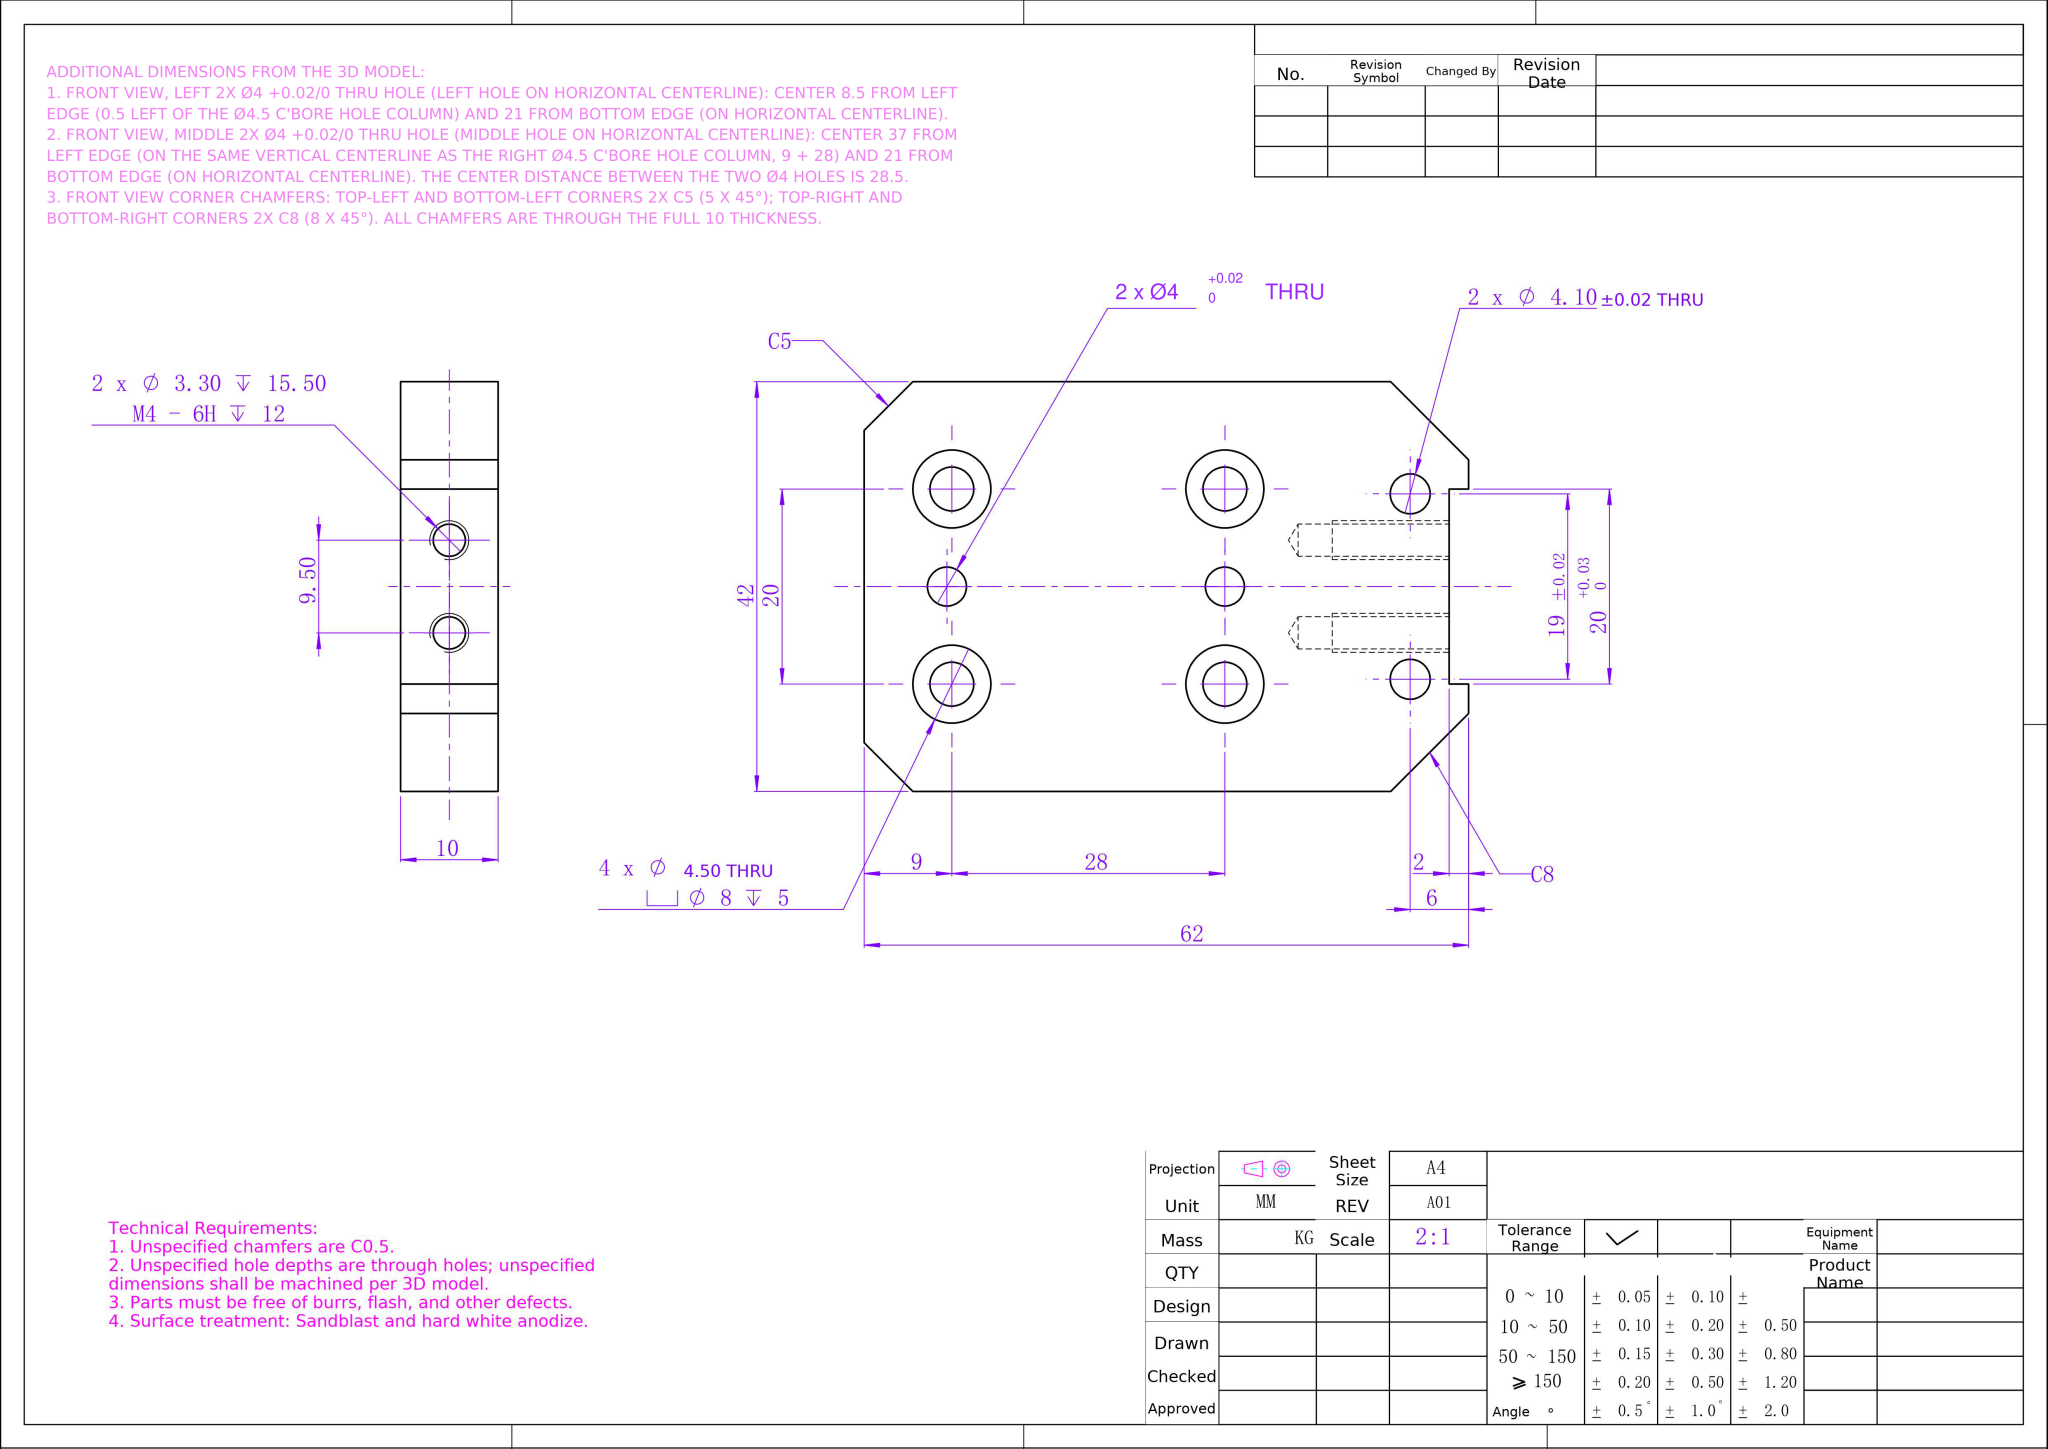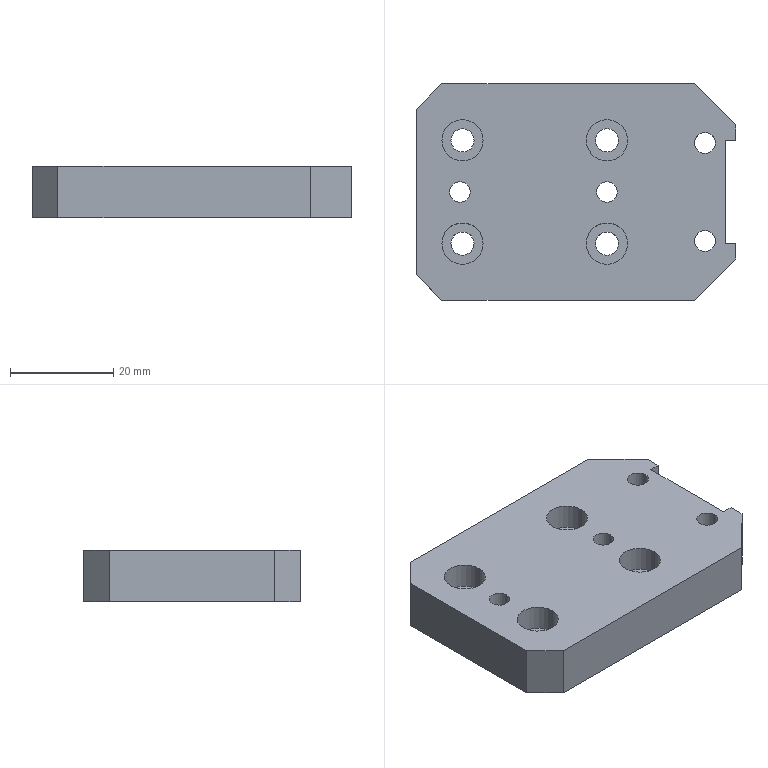Part | NX | mm | 1 solid | 50 faces | box 62 x 42 x 10 mm | volume 22640 mm3 | cylinder 28 | plane 18 | cone 4 | commonest cylinder face diameters 8 x8 4.5 x8 4 x4 4.1 x4 3.3 x4